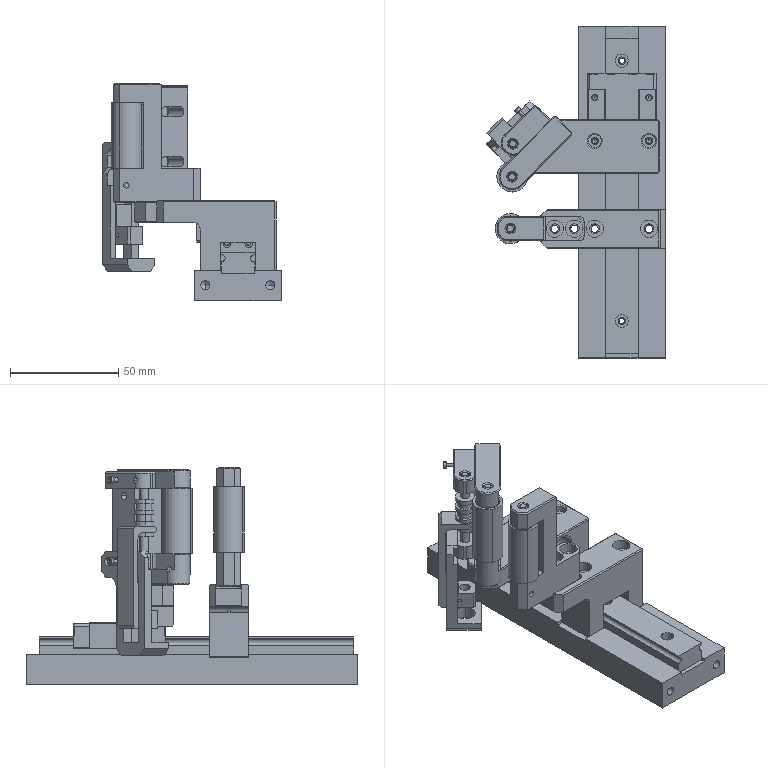Assembly | SolidWorks | mm | 19 component files | 19 solids | 779 faces | box 82.27 x 153 x 100.1 mm | volume 194225 mm3 | plane 424 | cylinder 250 | cone 98 | spline 7 | commonest cylinder face diameters 2.5 x28 4 x22 6 x16 8 x16 4.5 x16 3.5 x15 3 x14 3.3 x14
Bill of materials:
1-16 | 1 |  | Long straight bar of constant cross-section with four evenly spaced through holes on the top face and a rounded longitudinal groove along each side; the profile resembles a linear guide rail.
2-16 | 1 |  | Rectangular block with a channel underneath (inverted-U end profile), four holes in the top face, separate thinner end plates at both ends, and small recessed features on the end faces; it resembles a linear guide carriage block.
AdhesiveAssemblyFixedPlate | 1 |  | Long, flat rectangular plate with a shallow raised or stepped central strip area, a row of through holes of mixed sizes along the centerline, two extra holes on the sides near the middle, and threaded-looking or plain holes in one end face.
AdhesiveRoller | 2 |  | Plain cylindrical sleeve with a stepped axial bore: a larger counterbore at one end and a smaller through bore.
AdhesiveRollerFixedAxis | 2 |  | Slender solid cylindrical pin or rod with small chamfers on both ends.
GuideWheelFixedSeat | 1 |  | Bracket with a C-shaped side profile: a flat web plate with two projecting lugs that have rounded ends, each lug holding a vertical hole, and additional holes through the web and lugs.
hexagon socket head cap screws gb_PreviewCfg | 3 |  | Socket head cap screw-like fastener: a cylindrical head with a hexagonal socket recess and a plain cylindrical shank with a chamfered tip.
InnerAdjustmentBlock | 1 |  | Plate-like bracket with a stepped side profile and one large through hole; it has a hooked, C-shaped upper portion with rounded inner corners, stepped lower blocks, and small side holes.
InnerFineAdjustmentBlock | 1 |  | Clip-like plate part with an open rectangular window, an elongated slot at the top, a large round hole in a lower plate, a hooked flange with a rounded inner fillet, and chamfered corners.
LowerRollerFixedSeat | 1 |  | Rectangular block with a T/inverted-U side profile: a top bar with a filleted overhang on one side, a rectangular slot cut up from the bottom, and four through holes of two sizes along the top face plus a narrow groove.
LowerRollerMountingSeat | 1 |  | Stepped bracket shaped like a Z or offset: a tall vertical web joining a top tab with a hole to a lower base with two larger holes, an extra small hole at the lower left, and a small side hole.
TapeGuideRoller | 1 |  | Tubular cylindrical part with a through bore and four evenly spaced external annular flanges (ribs) along its length, giving a spool-like or grooved profile.
TapeGuideRollerAxis | 1 |  | Slender solid cylindrical pin/rod with small chamfers at both ends.
UpperRollerAxisSeat | 1 |  | C-shaped (U-profile) block bracket: a rectangular web with two parallel lugs coming off one side. Each lug has a rounded end with a small through hole. The web has two parallel transverse through bores, and there is a small hole near the base of one lug.
UpperRollerFixedSeat | 1 |  | Rectangular plate-like block with one chamfered (clipped) corner and four vertical holes: two plain holes and two counterbored holes. Underneath is a stepped lower section with one large transverse through bore.
Mates: